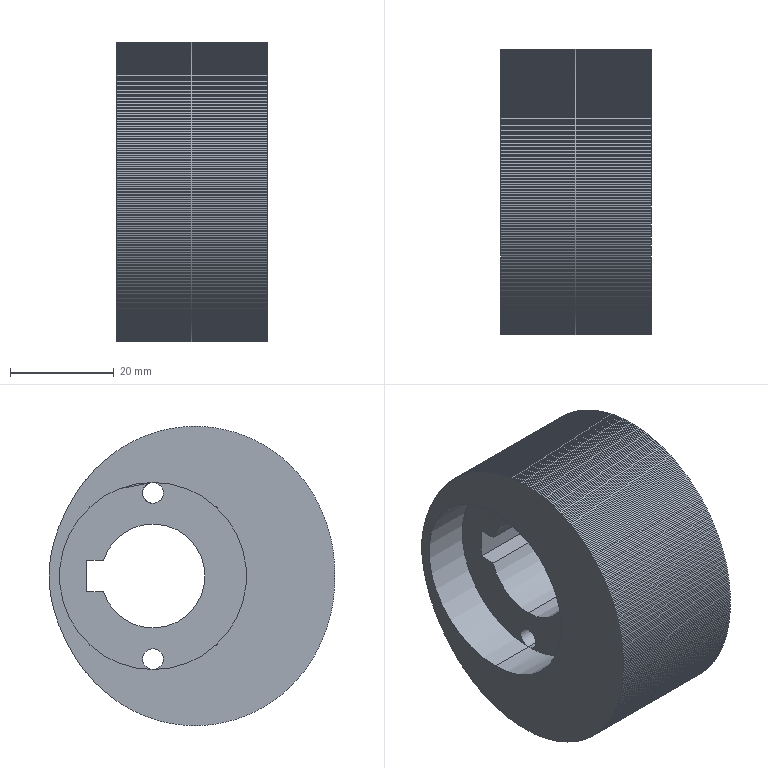Component | SolidWorks | CamGroup3-1_Cam6-1 | 1 solid | 644 faces | box 29 x 55 x 57.58 mm | volume 55505 mm3 | plane 635 | cylinder 9 | commonest cylinder face diameters 4 x4 20 x3 36 x2
build123d program:
from build123d import *

# Parameters (mm, degrees)
MODEL_R             = 2
BOSS_EXTRUDE1_DEPTH = 29
SKETCH2_R           = 18
CUT_EXTRUDE1_DEPTH  = 9


with BuildPart() as part:
    # Model → Boss-Extrude1 (new body)
    with BuildSketch(Plane.XY):
        Polygon((103.927, 136.86), (104.127, 136.859), (104.327, 136.856), (104.527, 136.851), (104.727, 136.844), (104.927, 136.835), (105.127, 136.825), (105.326, 136.812), (105.526, 136.798), (105.725, 136.782), (105.925, 136.764), (106.124, 136.745), (106.323, 136.724), (106.521, 136.701), (106.72, 136.676), (106.918, 136.65), (107.117, 136.622), (107.315, 136.593), (107.513, 136.562), (107.71, 136.529), (107.908, 136.495), (108.105, 136.46), (108.302, 136.423), (108.499, 136.384), (108.696, 136.344), (108.892, 136.303), (109.088, 136.26), (109.284, 136.215), (109.48, 136.17), (109.676, 136.123), (109.871, 136.074), (110.066, 136.024), (110.261, 135.973), (110.456, 135.92), (110.651, 135.866), (110.845, 135.811), (111.039, 135.754), (111.233, 135.696), (111.427, 135.637), (111.621, 135.576), (111.814, 135.514), (112.008, 135.451), (112.201, 135.387), (112.394, 135.321), (112.587, 135.254), (112.78, 135.185), (112.972, 135.115), (113.165, 135.044), (113.357, 134.972), (113.549, 134.898), (113.741, 134.823), (113.933, 134.747), (114.125, 134.67), (114.316, 134.591), (114.508, 134.51), (114.699, 134.429), (114.89, 134.346), (115.081, 134.262), (115.272, 134.176), (115.463, 134.089), (115.654, 134.001), (115.845, 133.911), (116.035, 133.82), (116.226, 133.727), (116.416, 133.633), (116.606, 133.538), (116.796, 133.441), (116.986, 133.343), (117.176, 133.243), (117.366, 133.142), (117.555, 133.039), (117.745, 132.935), (117.934, 132.829), (118.123, 132.722), (118.312, 132.613), (118.501, 132.503), (118.689, 132.391), (118.878, 132.278), (119.066, 132.163), (119.254, 132.046), (119.442, 131.927), (119.629, 131.807), (119.817, 131.686), (120.004, 131.562), (120.191, 131.437), (120.377, 131.31), (120.563, 131.182), (120.749, 131.052), (120.935, 130.92), (121.12, 130.786), (121.305, 130.65), (121.49, 130.513), (121.674, 130.373), (121.858, 130.232), (122.041, 130.089), (122.224, 129.944), (122.407, 129.797), (122.589, 129.648), (122.77, 129.498), (122.951, 129.345), (123.131, 129.19), (123.311, 129.034), (123.49, 128.875), (123.669, 128.715), (123.847, 128.552), (124.024, 128.387), (124.2, 128.221), (124.376, 128.052), (124.551, 127.881), (124.725, 127.708), (124.898, 127.533), (125.071, 127.356), (125.242, 127.177), (125.413, 126.995), (125.582, 126.812), (125.751, 126.626), (125.918, 126.438), (126.085, 126.249), (126.25, 126.056), (126.414, 125.862), (126.578, 125.666), (126.739, 125.467), (126.9, 125.266), (127.059, 125.063), (127.217, 124.858), (127.374, 124.65), (127.529, 124.441), (127.683, 124.229), (127.835, 124.015), (127.986, 123.799), (128.135, 123.58), (128.283, 123.36), (128.429, 123.137), (128.573, 122.912), (128.716, 122.684), (128.856, 122.455), (128.995, 122.224), (129.132, 121.99), (129.268, 121.754), (129.401, 121.516), (129.532, 121.276), (129.662, 121.034), (129.789, 120.789), (129.914, 120.543), (130.037, 120.294), (130.158, 120.044), (130.276, 119.791), (130.392, 119.536), (130.506, 119.28), (130.618, 119.021), (130.727, 118.76), (130.834, 118.498), (130.938, 118.233), (131.04, 117.966), (131.139, 117.698), (131.235, 117.428), (131.329, 117.156), (131.42, 116.882), (131.509, 116.606), (131.594, 116.328), (131.677, 116.049), (131.757, 115.768), (131.834, 115.485), (131.908, 115.201), (131.979, 114.915), (132.047, 114.628), (132.112, 114.339), (132.174, 114.048), (132.232, 113.756), (132.288, 113.463), (132.34, 113.168), (132.389, 112.872), (132.435, 112.574), (132.477, 112.276), (132.516, 111.976), (132.552, 111.674), (132.584, 111.372), (132.613, 111.069), (132.638, 110.764), (132.66, 110.459), (132.678, 110.152), (132.693, 109.845), (132.704, 109.536), (132.711, 109.227), (132.715, 108.917), (132.715, 108.606), (132.711, 108.295), (132.704, 107.983), (132.693, 107.671), (132.678, 107.358), (132.659, 107.044), (132.636, 106.73), (132.61, 106.416), (132.579, 106.101), (132.545, 105.786), (132.507, 105.471), (132.465, 105.156), (132.419, 104.84), (132.369, 104.525), (132.315, 104.21), (132.257, 103.894), (132.195, 103.579), (132.129, 103.264), (132.059, 102.95), (131.985, 102.635), (131.907, 102.321), (131.825, 102.008), (131.739, 101.695), (131.649, 101.382), (131.555, 101.071), (131.456, 100.759), (131.354, 100.449), (131.248, 100.139), (131.137, 99.831), (131.023, 99.523), (130.904, 99.216), (130.782, 98.91), (130.655, 98.605), (130.525, 98.302), (130.39, 97.999), (130.252, 97.698), (130.109, 97.399), (129.962, 97.1), (129.812, 96.804), (129.657, 96.508), (129.499, 96.215), (129.337, 95.923), (129.17, 95.632), (129, 95.344), (128.826, 95.057), (128.648, 94.772), (128.466, 94.489), (128.281, 94.208), (128.092, 93.929), (127.899, 93.652), (127.702, 93.378), (127.501, 93.105), (127.297, 92.835), (127.09, 92.568), (126.878, 92.302), (126.663, 92.039), (126.445, 91.779), (126.223, 91.521), (125.997, 91.266), (125.768, 91.013), (125.536, 90.763), (125.3, 90.516), (125.061, 90.271), (124.819, 90.03), (124.573, 89.791), (124.324, 89.555), (124.072, 89.323), (123.817, 89.093), (123.559, 88.866), (123.298, 88.642), (123.034, 88.422), (122.766, 88.205), (122.496, 87.991), (122.223, 87.78), (121.948, 87.573), (121.669, 87.369), (121.388, 87.168), (121.104, 86.971), (120.818, 86.777), (120.528, 86.586), (120.237, 86.399), (119.943, 86.216), (119.646, 86.036), (119.348, 85.86), (119.046, 85.688), (118.743, 85.519), (118.438, 85.354), (118.13, 85.192), (117.82, 85.034), (117.508, 84.88), (117.194, 84.73), (116.879, 84.583), (116.561, 84.441), (116.242, 84.302), (115.92, 84.167), (115.597, 84.035), (115.273, 83.908), (114.947, 83.784), (114.619, 83.664), (114.29, 83.549), (113.959, 83.437), (113.627, 83.328), (113.294, 83.224), (112.959, 83.124), (112.624, 83.028), (112.287, 82.935), (111.949, 82.846), (111.609, 82.762), (111.269, 82.681), (110.928, 82.604), (110.586, 82.531), (110.243, 82.461), (109.9, 82.396), (109.556, 82.334), (109.21, 82.277), (108.865, 82.223), (108.518, 82.173), (108.172, 82.126), (107.824, 82.084), (107.477, 82.045), (107.128, 82.01), (106.78, 81.979), (106.431, 81.951), (106.082, 81.927), (105.732, 81.907), (105.383, 81.89), (105.033, 81.877), (104.683, 81.868), (104.333, 81.862), (103.983, 81.86), (103.872, 81.86), (103.522, 81.862), (103.172, 81.868), (102.822, 81.877), (102.472, 81.89), (102.122, 81.907), (101.773, 81.927), (101.424, 81.951), (101.075, 81.979), (100.726, 82.01), (100.378, 82.045), (100.03, 82.084), (99.683, 82.126), (99.336, 82.173), (98.99, 82.223), (98.644, 82.277), (98.299, 82.334), (97.955, 82.396), (97.611, 82.461), (97.268, 82.531), (96.927, 82.604), (96.585, 82.681), (96.245, 82.762), (95.906, 82.846), (95.568, 82.935), (95.231, 83.028), (94.895, 83.124), (94.561, 83.224), (94.228, 83.328), (93.896, 83.437), (93.565, 83.549), (93.236, 83.664), (92.908, 83.784), (92.582, 83.908), (92.257, 84.035), (91.934, 84.167), (91.613, 84.302), (91.294, 84.441), (90.976, 84.583), (90.66, 84.73), (90.347, 84.88), (90.035, 85.034), (89.725, 85.192), (89.417, 85.354), (89.112, 85.519), (88.808, 85.688), (88.507, 85.86), (88.208, 86.036), (87.912, 86.216), (87.618, 86.399), (87.326, 86.586), (87.037, 86.777), (86.751, 86.971), (86.467, 87.168), (86.186, 87.369), (85.907, 87.573), (85.631, 87.78), (85.358, 87.991), (85.088, 88.205), (84.821, 88.422), (84.557, 88.642), (84.296, 88.866), (84.037, 89.093), (83.782, 89.323), (83.53, 89.555), (83.282, 89.791), (83.036, 90.03), (82.794, 90.271), (82.555, 90.516), (82.319, 90.763), (82.087, 91.013), (81.858, 91.266), (81.632, 91.521), (81.41, 91.779), (81.192, 92.039), (80.977, 92.302), (80.765, 92.568), (80.557, 92.835), (80.353, 93.105), (80.153, 93.378), (79.956, 93.652), (79.763, 93.929), (79.574, 94.208), (79.388, 94.489), (79.207, 94.772), (79.029, 95.057), (78.855, 95.344), (78.685, 95.632), (78.518, 95.923), (78.356, 96.215), (78.197, 96.508), (78.043, 96.804), (77.892, 97.1), (77.746, 97.399), (77.603, 97.698), (77.465, 97.999), (77.33, 98.302), (77.199, 98.605), (77.073, 98.91), (76.95, 99.216), (76.832, 99.523), (76.717, 99.831), (76.607, 100.139), (76.501, 100.449), (76.398, 100.759), (76.3, 101.071), (76.206, 101.382), (76.116, 101.695), (76.03, 102.008), (75.948, 102.321), (75.87, 102.635), (75.796, 102.95), (75.726, 103.264), (75.66, 103.579), (75.598, 103.894), (75.54, 104.21), (75.486, 104.525), (75.436, 104.84), (75.39, 105.156), (75.348, 105.471), (75.31, 105.786), (75.275, 106.101), (75.245, 106.416), (75.218, 106.73), (75.196, 107.044), (75.177, 107.358), (75.162, 107.671), (75.151, 107.983), (75.143, 108.295), (75.14, 108.606), (75.14, 108.917), (75.143, 109.227), (75.151, 109.536), (75.162, 109.845), (75.176, 110.152), (75.195, 110.459), (75.216, 110.764), (75.242, 111.069), (75.271, 111.372), (75.303, 111.674), (75.338, 111.976), (75.378, 112.276), (75.42, 112.574), (75.466, 112.872), (75.515, 113.168), (75.567, 113.463), (75.623, 113.756), (75.681, 114.048), (75.743, 114.339), (75.808, 114.628), (75.876, 114.915), (75.947, 115.201), (76.021, 115.485), (76.098, 115.768), (76.178, 116.049), (76.261, 116.328), (76.346, 116.606), (76.435, 116.882), (76.526, 117.156), (76.619, 117.428), (76.716, 117.698), (76.815, 117.966), (76.917, 118.233), (77.021, 118.498), (77.128, 118.76), (77.237, 119.021), (77.348, 119.28), (77.462, 119.536), (77.579, 119.791), (77.697, 120.044), (77.818, 120.294), (77.941, 120.543), (78.066, 120.789), (78.193, 121.034), (78.322, 121.276), (78.454, 121.516), (78.587, 121.754), (78.722, 121.99), (78.859, 122.224), (78.998, 122.455), (79.139, 122.684), (79.282, 122.912), (79.426, 123.137), (79.572, 123.36), (79.72, 123.58), (79.869, 123.799), (80.02, 124.015), (80.172, 124.229), (80.326, 124.441), (80.481, 124.65), (80.638, 124.858), (80.795, 125.063), (80.955, 125.266), (81.115, 125.467), (81.277, 125.666), (81.44, 125.862), (81.605, 126.056), (81.77, 126.249), (81.936, 126.438), (82.104, 126.626), (82.273, 126.812), (82.442, 126.995), (82.613, 127.177), (82.784, 127.356), (82.957, 127.533), (83.13, 127.708), (83.304, 127.881), (83.479, 128.052), (83.654, 128.221), (83.831, 128.387), (84.008, 128.552), (84.186, 128.715), (84.364, 128.875), (84.544, 129.034), (84.723, 129.19), (84.904, 129.345), (85.085, 129.498), (85.266, 129.648), (85.448, 129.797), (85.63, 129.944), (85.813, 130.089), (85.997, 130.232), (86.181, 130.373), (86.365, 130.513), (86.549, 130.65), (86.734, 130.786), (86.92, 130.92), (87.105, 131.052), (87.291, 131.182), (87.478, 131.31), (87.664, 131.437), (87.851, 131.562), (88.038, 131.686), (88.225, 131.807), (88.413, 131.927), (88.601, 132.046), (88.789, 132.163), (88.977, 132.278), (89.165, 132.391), (89.354, 132.503), (89.543, 132.613), (89.732, 132.722), (89.921, 132.829), (90.11, 132.935), (90.299, 133.039), (90.489, 133.142), (90.679, 133.243), (90.869, 133.343), (91.058, 133.441), (91.249, 133.538), (91.439, 133.633), (91.629, 133.727), (91.819, 133.82), (92.01, 133.911), (92.201, 134.001), (92.391, 134.089), (92.582, 134.176), (92.773, 134.262), (92.964, 134.346), (93.156, 134.429), (93.347, 134.51), (93.539, 134.591), (93.73, 134.67), (93.922, 134.747), (94.114, 134.823), (94.306, 134.898), (94.498, 134.972), (94.69, 135.044), (94.883, 135.115), (95.075, 135.185), (95.268, 135.254), (95.461, 135.321), (95.654, 135.387), (95.847, 135.451), (96.04, 135.514), (96.234, 135.576), (96.428, 135.637), (96.621, 135.696), (96.815, 135.754), (97.01, 135.811), (97.204, 135.866), (97.399, 135.92), (97.593, 135.973), (97.789, 136.024), (97.984, 136.074), (98.179, 136.123), (98.375, 136.17), (98.571, 136.215), (98.767, 136.26), (98.963, 136.303), (99.159, 136.344), (99.356, 136.384), (99.553, 136.423), (99.75, 136.46), (99.947, 136.495), (100.144, 136.529), (100.342, 136.562), (100.54, 136.593), (100.738, 136.622), (100.936, 136.65), (101.135, 136.676), (101.333, 136.701), (101.532, 136.724), (101.731, 136.745), (101.93, 136.764), (102.13, 136.782), (102.329, 136.798), (102.528, 136.812), (102.728, 136.825), (102.928, 136.835), (103.128, 136.844), (103.327, 136.851), (103.527, 136.856), (103.727, 136.859), align=None)
        with Locations(Location((87.927, 116.862, 0), (0, 0, 180))):
            Circle(MODEL_R, mode=Mode.SUBTRACT)
        with Locations(Location((119.927, 116.862, 0), (0, 0, 180))):
            Circle(MODEL_R, mode=Mode.SUBTRACT)
        with BuildLine():
            Line((106.927, 129.646), (106.927, 126.401))
            ThreePointArc((106.927, 126.401), (103.927, 106.862), (100.927, 126.401))
            Line((100.927, 126.401), (100.927, 129.646))
            Line((100.927, 129.646), (106.927, 129.646))
        make_face(mode=Mode.SUBTRACT)
    extrude(amount=BOSS_EXTRUDE1_DEPTH)

    # Sketch2 → Cut-Extrude1 (cut)
    with BuildSketch(Plane.XY.offset(29)):
        with Locations((103.927, 116.862)):
            Circle(SKETCH2_R)
    extrude(amount=-CUT_EXTRUDE1_DEPTH, mode=Mode.SUBTRACT)


solid = part.part

# Placed as in the assembly
solid = solid.moved(Location((-104.938, -101.746, 245.073), (0, -90, 0)))